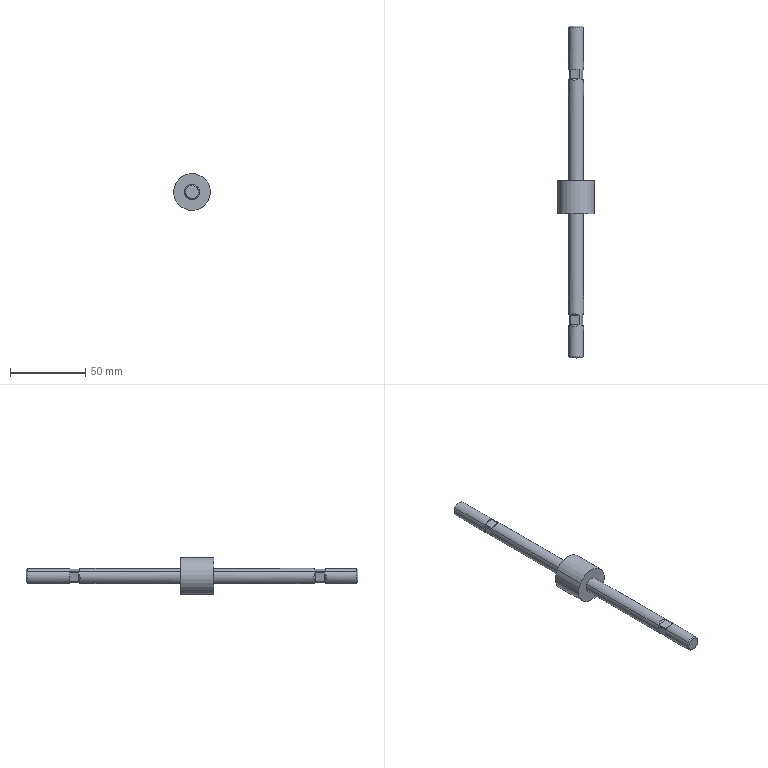Component | SolidWorks | MACJ25x25-10S-Rod-1_MACJ25x25-10S-Rod-1 | 1 solid | 38 faces | box 24.5 x 221 x 24.5 mm | volume 25761 mm3 | plane 28 | cylinder 6 | cone 4 | commonest cylinder face diameters 10 x4 24.5 x2
STEP:
#1=CARTESIAN_POINT('',(-0.3117,9.81,-6.329));
#2=VERTEX_POINT('',#1);
#3=CARTESIAN_POINT('',(-0.0297,9.81,-6.507));
#4=VERTEX_POINT('',#3);
#5=CARTESIAN_POINT('',(-0.1707,9.81,-6.418));
#6=DIRECTION('',(0.,-1.,-0.));
#7=DIRECTION('',(-0.846,0.,0.5333));
#8=AXIS2_PLACEMENT_3D('',#5,#6,#7);
#9=CIRCLE('',#8,0.1667);
#10=EDGE_CURVE('',#2,#4,#9,.T.);
#11=ORIENTED_EDGE('',*,*,#10,.T.);
#12=CARTESIAN_POINT('',(-0.00415,9.78,-6.523));
#13=VERTEX_POINT('',#12);
#14=CARTESIAN_POINT('',(-0.0297,9.81,-6.507));
#15=DIRECTION('',(0.5982,-0.7071,-0.3771));
#16=VECTOR('',#15,39.37);
#17=LINE('',#14,#16);
#18=EDGE_CURVE('',#4,#13,#17,.T.);
#19=ORIENTED_EDGE('',*,*,#18,.T.);
#20=CARTESIAN_POINT('',(-0.3372,9.78,-6.313));
#21=VERTEX_POINT('',#20);
#22=CARTESIAN_POINT('',(-0.1707,9.78,-6.418));
#23=DIRECTION('',(0.,-1.,-0.));
#24=DIRECTION('',(-0.846,0.,0.5333));
#25=AXIS2_PLACEMENT_3D('',#22,#23,#24);
#26=CIRCLE('',#25,0.1969);
#27=EDGE_CURVE('',#21,#13,#26,.T.);
#28=ORIENTED_EDGE('',*,*,#27,.F.);
#29=CARTESIAN_POINT('',(-0.3117,9.81,-6.329));
#30=DIRECTION('',(-0.5982,-0.7071,0.3771));
#31=VECTOR('',#30,39.37);
#32=LINE('',#29,#31);
#33=EDGE_CURVE('',#2,#21,#32,.T.);
#34=ORIENTED_EDGE('',*,*,#33,.F.);
#35=EDGE_LOOP('',(#11,#19,#28,#34));
#36=FACE_OUTER_BOUND('',#35,.T.);
#37=CARTESIAN_POINT('',(-0.1707,9.81,-6.418));
#38=DIRECTION('',(0.,-1.,-0.));
#39=DIRECTION('',(-0.846,0.,0.5333));
#40=AXIS2_PLACEMENT_3D('',#37,#38,#39);
#41=CONICAL_SURFACE('',#40,0.1667,0.7854);
#42=ADVANCED_FACE('',(#36),#41,.T.);
#43=CARTESIAN_POINT('',(-0.2981,8.432,-6.568));
#44=VERTEX_POINT('',#43);
#45=CARTESIAN_POINT('',(-0.2981,8.668,-6.568));
#46=VERTEX_POINT('',#45);
#47=CARTESIAN_POINT('',(-0.2981,9.81,-6.568));
#48=DIRECTION('',(-0.,1.,0.));
#49=VECTOR('',#48,39.37);
#50=LINE('',#47,#49);
#51=EDGE_CURVE('',#44,#46,#50,.T.);
#52=ORIENTED_EDGE('',*,*,#51,.T.);
#53=CARTESIAN_POINT('',(-0.3504,8.668,-6.338));
#54=VERTEX_POINT('',#53);
#55=CARTESIAN_POINT('',(-0.1707,8.668,-6.418));
#56=DIRECTION('',(-0.,1.,0.));
#57=DIRECTION('',(0.846,0.,-0.5333));
#58=AXIS2_PLACEMENT_3D('',#55,#56,#57);
#59=CIRCLE('',#58,0.1969);
#60=EDGE_CURVE('',#46,#54,#59,.T.);
#61=ORIENTED_EDGE('',*,*,#60,.T.);
#62=CARTESIAN_POINT('',(-0.3504,8.432,-6.338));
#63=VERTEX_POINT('',#62);
#64=CARTESIAN_POINT('',(-0.3504,9.81,-6.338));
#65=DIRECTION('',(0.,-1.,-0.));
#66=VECTOR('',#65,39.37);
#67=LINE('',#64,#66);
#68=EDGE_CURVE('',#54,#63,#67,.T.);
#69=ORIENTED_EDGE('',*,*,#68,.T.);
#70=CARTESIAN_POINT('',(-0.3504,8.432,-6.338));
#71=CARTESIAN_POINT('',(-0.3875,8.377,-6.42));
#72=CARTESIAN_POINT('',(-0.3674,8.377,-6.509));
#73=CARTESIAN_POINT('',(-0.2981,8.432,-6.568));
#74=(BOUNDED_CURVE()B_SPLINE_CURVE(3,(#70,#71,#72,#73),.UNSPECIFIED.,.F.,.T.)B_SPLINE_CURVE_WITH_KNOTS((4,4),(5.64,6.927),.UNSPECIFIED.)CURVE()GEOMETRIC_REPRESENTATION_ITEM()RATIONAL_B_SPLINE_CURVE((1.,0.8667,0.8667,1.))REPRESENTATION_ITEM(''));
#75=EDGE_CURVE('',#63,#44,#74,.T.);
#76=ORIENTED_EDGE('',*,*,#75,.T.);
#77=EDGE_LOOP('',(#52,#61,#69,#76));
#78=FACE_BOUND('',#77,.T.);
#79=CARTESIAN_POINT('',(-0.02067,8.432,-6.545));
#80=VERTEX_POINT('',#79);
#81=CARTESIAN_POINT('',(-0.02067,8.668,-6.545));
#82=VERTEX_POINT('',#81);
#83=CARTESIAN_POINT('',(-0.02067,9.81,-6.545));
#84=DIRECTION('',(-0.,1.,0.));
#85=VECTOR('',#84,39.37);
#86=LINE('',#83,#85);
#87=EDGE_CURVE('',#80,#82,#86,.T.);
#88=ORIENTED_EDGE('',*,*,#87,.T.);
#89=CARTESIAN_POINT('',(-0.251,8.668,-6.598));
#90=VERTEX_POINT('',#89);
#91=CARTESIAN_POINT('',(-0.1707,8.668,-6.418));
#92=DIRECTION('',(-0.,1.,0.));
#93=DIRECTION('',(0.846,0.,-0.5333));
#94=AXIS2_PLACEMENT_3D('',#91,#92,#93);
#95=CIRCLE('',#94,0.1969);
#96=EDGE_CURVE('',#82,#90,#95,.T.);
#97=ORIENTED_EDGE('',*,*,#96,.T.);
#98=CARTESIAN_POINT('',(-0.251,8.432,-6.598));
#99=VERTEX_POINT('',#98);
#100=CARTESIAN_POINT('',(-0.251,9.81,-6.598));
#101=DIRECTION('',(0.,-1.,-0.));
#102=VECTOR('',#101,39.37);
#103=LINE('',#100,#102);
#104=EDGE_CURVE('',#90,#99,#103,.T.);
#105=ORIENTED_EDGE('',*,*,#104,.T.);
#106=CARTESIAN_POINT('',(-0.251,8.432,-6.598));
#107=CARTESIAN_POINT('',(-0.1681,8.377,-6.635));
#108=CARTESIAN_POINT('',(-0.0795,8.377,-6.615));
#109=CARTESIAN_POINT('',(-0.02067,8.432,-6.545));
#110=(BOUNDED_CURVE()B_SPLINE_CURVE(3,(#106,#107,#108,#109),.UNSPECIFIED.,.F.,.F.)B_SPLINE_CURVE_WITH_KNOTS((4,4),(5.64,6.927),.UNSPECIFIED.)CURVE()GEOMETRIC_REPRESENTATION_ITEM()RATIONAL_B_SPLINE_CURVE((1.,0.8667,0.8667,1.))REPRESENTATION_ITEM(''));
#111=EDGE_CURVE('',#99,#80,#110,.T.);
#112=ORIENTED_EDGE('',*,*,#111,.T.);
#113=EDGE_LOOP('',(#88,#97,#105,#112));
#114=FACE_BOUND('',#113,.T.);
#115=ORIENTED_EDGE('',*,*,#27,.T.);
#116=CARTESIAN_POINT('',(-0.00415,5.755,-6.523));
#117=VERTEX_POINT('',#116);
#118=CARTESIAN_POINT('',(-0.00415,9.81,-6.523));
#119=DIRECTION('',(0.,-1.,-0.));
#120=VECTOR('',#119,39.37);
#121=LINE('',#118,#120);
#122=EDGE_CURVE('',#13,#117,#121,.T.);
#123=ORIENTED_EDGE('',*,*,#122,.T.);
#124=CARTESIAN_POINT('',(-0.3372,5.755,-6.313));
#125=VERTEX_POINT('',#124);
#126=CARTESIAN_POINT('',(-0.1707,5.755,-6.418));
#127=DIRECTION('',(0.,-1.,-0.));
#128=DIRECTION('',(-0.846,0.,0.5333));
#129=AXIS2_PLACEMENT_3D('',#126,#127,#128);
#130=CIRCLE('',#129,0.1969);
#131=EDGE_CURVE('',#125,#117,#130,.T.);
#132=ORIENTED_EDGE('',*,*,#131,.F.);
#133=CARTESIAN_POINT('',(-0.3372,9.81,-6.313));
#134=DIRECTION('',(0.,-1.,-0.));
#135=VECTOR('',#134,39.37);
#136=LINE('',#133,#135);
#137=EDGE_CURVE('',#21,#125,#136,.T.);
#138=ORIENTED_EDGE('',*,*,#137,.F.);
#139=EDGE_LOOP('',(#115,#123,#132,#138));
#140=FACE_OUTER_BOUND('',#139,.T.);
#141=CARTESIAN_POINT('',(-0.1707,9.81,-6.418));
#142=DIRECTION('',(0.,-1.,-0.));
#143=DIRECTION('',(-0.846,0.,0.5333));
#144=AXIS2_PLACEMENT_3D('',#141,#142,#143);
#145=CYLINDRICAL_SURFACE('',#144,0.1969);
#146=ADVANCED_FACE('',(#78,#114,#140),#145,.T.);
#147=CARTESIAN_POINT('',(-0.5787,5.755,-6.161));
#148=VERTEX_POINT('',#147);
#149=CARTESIAN_POINT('',(0.2373,5.755,-6.675));
#150=VERTEX_POINT('',#149);
#151=CARTESIAN_POINT('',(-0.1707,5.755,-6.418));
#152=DIRECTION('',(0.,-1.,-0.));
#153=DIRECTION('',(-0.846,0.,0.5333));
#154=AXIS2_PLACEMENT_3D('',#151,#152,#153);
#155=CIRCLE('',#154,0.4823);
#156=EDGE_CURVE('',#148,#150,#155,.T.);
#157=ORIENTED_EDGE('',*,*,#156,.T.);
#158=CARTESIAN_POINT('',(0.2373,4.889,-6.675));
#159=VERTEX_POINT('',#158);
#160=CARTESIAN_POINT('',(0.2373,9.81,-6.675));
#161=DIRECTION('',(0.,-1.,-0.));
#162=VECTOR('',#161,39.37);
#163=LINE('',#160,#162);
#164=EDGE_CURVE('',#150,#159,#163,.T.);
#165=ORIENTED_EDGE('',*,*,#164,.T.);
#166=CARTESIAN_POINT('',(-0.5787,4.889,-6.161));
#167=VERTEX_POINT('',#166);
#168=CARTESIAN_POINT('',(-0.1707,4.889,-6.418));
#169=DIRECTION('',(0.,-1.,-0.));
#170=DIRECTION('',(-0.846,0.,0.5333));
#171=AXIS2_PLACEMENT_3D('',#168,#169,#170);
#172=CIRCLE('',#171,0.4823);
#173=EDGE_CURVE('',#167,#159,#172,.T.);
#174=ORIENTED_EDGE('',*,*,#173,.F.);
#175=CARTESIAN_POINT('',(-0.5787,9.81,-6.161));
#176=DIRECTION('',(0.,-1.,-0.));
#177=VECTOR('',#176,39.37);
#178=LINE('',#175,#177);
#179=EDGE_CURVE('',#148,#167,#178,.T.);
#180=ORIENTED_EDGE('',*,*,#179,.F.);
#181=EDGE_LOOP('',(#157,#165,#174,#180));
#182=FACE_OUTER_BOUND('',#181,.T.);
#183=CARTESIAN_POINT('',(-0.1707,9.81,-6.418));
#184=DIRECTION('',(0.,-1.,-0.));
#185=DIRECTION('',(-0.846,0.,0.5333));
#186=AXIS2_PLACEMENT_3D('',#183,#184,#185);
#187=CYLINDRICAL_SURFACE('',#186,0.4823);
#188=ADVANCED_FACE('',(#182),#187,.T.);
#189=CARTESIAN_POINT('',(-0.2981,1.975,-6.568));
#190=VERTEX_POINT('',#189);
#191=CARTESIAN_POINT('',(-0.2981,2.227,-6.568));
#192=VERTEX_POINT('',#191);
#193=CARTESIAN_POINT('',(-0.2981,9.81,-6.568));
#194=DIRECTION('',(-0.,1.,0.));
#195=VECTOR('',#194,39.37);
#196=LINE('',#193,#195);
#197=EDGE_CURVE('',#190,#192,#196,.T.);
#198=ORIENTED_EDGE('',*,*,#197,.T.);
#199=CARTESIAN_POINT('',(-0.3504,2.227,-6.338));
#200=VERTEX_POINT('',#199);
#201=CARTESIAN_POINT('',(-0.2981,2.227,-6.568));
#202=CARTESIAN_POINT('',(-0.3674,2.282,-6.509));
#203=CARTESIAN_POINT('',(-0.3875,2.282,-6.42));
#204=CARTESIAN_POINT('',(-0.3504,2.227,-6.338));
#205=(BOUNDED_CURVE()B_SPLINE_CURVE(3,(#201,#202,#203,#204),.UNSPECIFIED.,.F.,.T.)B_SPLINE_CURVE_WITH_KNOTS((4,4),(2.498,3.785),.UNSPECIFIED.)CURVE()GEOMETRIC_REPRESENTATION_ITEM()RATIONAL_B_SPLINE_CURVE((1.,0.8667,0.8667,1.))REPRESENTATION_ITEM(''));
#206=EDGE_CURVE('',#192,#200,#205,.T.);
#207=ORIENTED_EDGE('',*,*,#206,.T.);
#208=CARTESIAN_POINT('',(-0.3504,1.975,-6.338));
#209=VERTEX_POINT('',#208);
#210=CARTESIAN_POINT('',(-0.3504,9.81,-6.338));
#211=DIRECTION('',(0.,-1.,-0.));
#212=VECTOR('',#211,39.37);
#213=LINE('',#210,#212);
#214=EDGE_CURVE('',#200,#209,#213,.T.);
#215=ORIENTED_EDGE('',*,*,#214,.T.);
#216=CARTESIAN_POINT('',(-0.3504,1.975,-6.338));
#217=CARTESIAN_POINT('',(-0.3875,1.921,-6.42));
#218=CARTESIAN_POINT('',(-0.3674,1.921,-6.509));
#219=CARTESIAN_POINT('',(-0.2981,1.975,-6.568));
#220=(BOUNDED_CURVE()B_SPLINE_CURVE(3,(#216,#217,#218,#219),.UNSPECIFIED.,.F.,.F.)B_SPLINE_CURVE_WITH_KNOTS((4,4),(5.64,6.927),.UNSPECIFIED.)CURVE()GEOMETRIC_REPRESENTATION_ITEM()RATIONAL_B_SPLINE_CURVE((1.,0.8667,0.8667,1.))REPRESENTATION_ITEM(''));
#221=EDGE_CURVE('',#209,#190,#220,.T.);
#222=ORIENTED_EDGE('',*,*,#221,.T.);
#223=EDGE_LOOP('',(#198,#207,#215,#222));
#224=FACE_BOUND('',#223,.T.);
#225=CARTESIAN_POINT('',(-0.02067,1.975,-6.545));
#226=VERTEX_POINT('',#225);
#227=CARTESIAN_POINT('',(-0.02067,2.227,-6.545));
#228=VERTEX_POINT('',#227);
#229=CARTESIAN_POINT('',(-0.02067,9.81,-6.545));
#230=DIRECTION('',(-0.,1.,0.));
#231=VECTOR('',#230,39.37);
#232=LINE('',#229,#231);
#233=EDGE_CURVE('',#226,#228,#232,.T.);
#234=ORIENTED_EDGE('',*,*,#233,.T.);
#235=CARTESIAN_POINT('',(-0.251,2.227,-6.598));
#236=VERTEX_POINT('',#235);
#237=CARTESIAN_POINT('',(-0.02067,2.227,-6.545));
#238=CARTESIAN_POINT('',(-0.0795,2.282,-6.615));
#239=CARTESIAN_POINT('',(-0.1681,2.282,-6.635));
#240=CARTESIAN_POINT('',(-0.251,2.227,-6.598));
#241=(BOUNDED_CURVE()B_SPLINE_CURVE(3,(#237,#238,#239,#240),.UNSPECIFIED.,.F.,.T.)B_SPLINE_CURVE_WITH_KNOTS((4,4),(2.498,3.785),.UNSPECIFIED.)CURVE()GEOMETRIC_REPRESENTATION_ITEM()RATIONAL_B_SPLINE_CURVE((1.,0.8667,0.8667,1.))REPRESENTATION_ITEM(''));
#242=EDGE_CURVE('',#228,#236,#241,.T.);
#243=ORIENTED_EDGE('',*,*,#242,.T.);
#244=CARTESIAN_POINT('',(-0.251,1.975,-6.598));
#245=VERTEX_POINT('',#244);
#246=CARTESIAN_POINT('',(-0.251,9.81,-6.598));
#247=DIRECTION('',(0.,-1.,-0.));
#248=VECTOR('',#247,39.37);
#249=LINE('',#246,#248);
#250=EDGE_CURVE('',#236,#245,#249,.T.);
#251=ORIENTED_EDGE('',*,*,#250,.T.);
#252=CARTESIAN_POINT('',(-0.251,1.975,-6.598));
#253=CARTESIAN_POINT('',(-0.1681,1.921,-6.635));
#254=CARTESIAN_POINT('',(-0.0795,1.921,-6.615));
#255=CARTESIAN_POINT('',(-0.02067,1.975,-6.545));
#256=(BOUNDED_CURVE()B_SPLINE_CURVE(3,(#252,#253,#254,#255),.UNSPECIFIED.,.F.,.T.)B_SPLINE_CURVE_WITH_KNOTS((4,4),(5.64,6.927),.UNSPECIFIED.)CURVE()GEOMETRIC_REPRESENTATION_ITEM()RATIONAL_B_SPLINE_CURVE((1.,0.8667,0.8667,1.))REPRESENTATION_ITEM(''));
#257=EDGE_CURVE('',#245,#226,#256,.T.);
#258=ORIENTED_EDGE('',*,*,#257,.T.);
#259=EDGE_LOOP('',(#234,#243,#251,#258));
#260=FACE_BOUND('',#259,.T.);
#261=CARTESIAN_POINT('',(-0.3372,4.889,-6.313));
#262=VERTEX_POINT('',#261);
#263=CARTESIAN_POINT('',(-0.00415,4.889,-6.523));
#264=VERTEX_POINT('',#263);
#265=CARTESIAN_POINT('',(-0.1707,4.889,-6.418));
#266=DIRECTION('',(0.,-1.,-0.));
#267=DIRECTION('',(-0.846,0.,0.5333));
#268=AXIS2_PLACEMENT_3D('',#265,#266,#267);
#269=CIRCLE('',#268,0.1969);
#270=EDGE_CURVE('',#262,#264,#269,.T.);
#271=ORIENTED_EDGE('',*,*,#270,.T.);
#272=CARTESIAN_POINT('',(-0.00415,1.139,-6.523));
#273=VERTEX_POINT('',#272);
#274=CARTESIAN_POINT('',(-0.00415,9.81,-6.523));
#275=DIRECTION('',(0.,-1.,-0.));
#276=VECTOR('',#275,39.37);
#277=LINE('',#274,#276);
#278=EDGE_CURVE('',#264,#273,#277,.T.);
#279=ORIENTED_EDGE('',*,*,#278,.T.);
#280=CARTESIAN_POINT('',(-0.3372,1.139,-6.313));
#281=VERTEX_POINT('',#280);
#282=CARTESIAN_POINT('',(-0.1707,1.139,-6.418));
#283=DIRECTION('',(0.,-1.,-0.));
#284=DIRECTION('',(-0.846,0.,0.5333));
#285=AXIS2_PLACEMENT_3D('',#282,#283,#284);
#286=CIRCLE('',#285,0.1969);
#287=EDGE_CURVE('',#281,#273,#286,.T.);
#288=ORIENTED_EDGE('',*,*,#287,.F.);
#289=CARTESIAN_POINT('',(-0.3372,9.81,-6.313));
#290=DIRECTION('',(0.,-1.,-0.));
#291=VECTOR('',#290,39.37);
#292=LINE('',#289,#291);
#293=EDGE_CURVE('',#262,#281,#292,.T.);
#294=ORIENTED_EDGE('',*,*,#293,.F.);
#295=EDGE_LOOP('',(#271,#279,#288,#294));
#296=FACE_OUTER_BOUND('',#295,.T.);
#297=CARTESIAN_POINT('',(-0.1707,9.81,-6.418));
#298=DIRECTION('',(0.,-1.,-0.));
#299=DIRECTION('',(-0.846,0.,0.5333));
#300=AXIS2_PLACEMENT_3D('',#297,#298,#299);
#301=CYLINDRICAL_SURFACE('',#300,0.1969);
#302=ADVANCED_FACE('',(#224,#260,#296),#301,.T.);
#303=CARTESIAN_POINT('',(-0.3117,1.109,-6.329));
#304=VERTEX_POINT('',#303);
#305=CARTESIAN_POINT('',(-0.0297,1.109,-6.507));
#306=VERTEX_POINT('',#305);
#307=CARTESIAN_POINT('',(-0.1707,1.109,-6.418));
#308=DIRECTION('',(0.,-1.,-0.));
#309=DIRECTION('',(-0.846,0.,0.5333));
#310=AXIS2_PLACEMENT_3D('',#307,#308,#309);
#311=CIRCLE('',#310,0.1667);
#312=EDGE_CURVE('',#304,#306,#311,.T.);
#313=ORIENTED_EDGE('',*,*,#312,.F.);
#314=CARTESIAN_POINT('',(-0.3372,1.139,-6.313));
#315=DIRECTION('',(-0.5982,0.7071,0.3771));
#316=VECTOR('',#315,39.37);
#317=LINE('',#314,#316);
#318=EDGE_CURVE('',#304,#281,#317,.T.);
#319=ORIENTED_EDGE('',*,*,#318,.T.);
#320=ORIENTED_EDGE('',*,*,#287,.T.);
#321=CARTESIAN_POINT('',(-0.00415,1.139,-6.523));
#322=DIRECTION('',(0.5982,0.7071,-0.3771));
#323=VECTOR('',#322,39.37);
#324=LINE('',#321,#323);
#325=EDGE_CURVE('',#306,#273,#324,.T.);
#326=ORIENTED_EDGE('',*,*,#325,.F.);
#327=EDGE_LOOP('',(#313,#319,#320,#326));
#328=FACE_OUTER_BOUND('',#327,.T.);
#329=CARTESIAN_POINT('',(-0.1707,1.139,-6.418));
#330=DIRECTION('',(-0.,1.,0.));
#331=DIRECTION('',(0.846,0.,-0.5333));
#332=AXIS2_PLACEMENT_3D('',#329,#330,#331);
#333=CONICAL_SURFACE('',#332,0.1969,0.7854);
#334=ADVANCED_FACE('',(#328),#333,.T.);
#335=CARTESIAN_POINT('',(-0.1707,1.109,-6.418));
#336=DIRECTION('',(0.,-1.,-0.));
#337=DIRECTION('',(-0.846,0.,0.5333));
#338=AXIS2_PLACEMENT_3D('',#335,#336,#337);
#339=CIRCLE('',#338,0.1667);
#340=EDGE_CURVE('',#306,#304,#339,.T.);
#341=ORIENTED_EDGE('',*,*,#340,.T.);
#342=ORIENTED_EDGE('',*,*,#312,.T.);
#343=EDGE_LOOP('',(#341,#342));
#344=FACE_OUTER_BOUND('',#343,.T.);
#345=CARTESIAN_POINT('',(-0.1707,1.109,-6.418));
#346=DIRECTION('',(-0.,1.,0.));
#347=DIRECTION('',(0.846,0.,-0.5333));
#348=AXIS2_PLACEMENT_3D('',#345,#346,#347);
#349=PLANE('',#348);
#350=ADVANCED_FACE('',(#344),#349,.F.);
#351=ORIENTED_EDGE('',*,*,#318,.F.);
#352=ORIENTED_EDGE('',*,*,#340,.F.);
#353=ORIENTED_EDGE('',*,*,#325,.T.);
#354=CARTESIAN_POINT('',(-0.1707,1.139,-6.418));
#355=DIRECTION('',(0.,-1.,-0.));
#356=DIRECTION('',(-0.846,0.,0.5333));
#357=AXIS2_PLACEMENT_3D('',#354,#355,#356);
#358=CIRCLE('',#357,0.1969);
#359=EDGE_CURVE('',#273,#281,#358,.T.);
#360=ORIENTED_EDGE('',*,*,#359,.T.);
#361=EDGE_LOOP('',(#351,#352,#353,#360));
#362=FACE_OUTER_BOUND('',#361,.T.);
#363=CARTESIAN_POINT('',(-0.1707,1.139,-6.418));
#364=DIRECTION('',(-0.,1.,0.));
#365=DIRECTION('',(0.846,0.,-0.5333));
#366=AXIS2_PLACEMENT_3D('',#363,#364,#365);
#367=CONICAL_SURFACE('',#366,0.1969,0.7854);
#368=ADVANCED_FACE('',(#362),#367,.T.);
#369=ORIENTED_EDGE('',*,*,#278,.F.);
#370=CARTESIAN_POINT('',(-0.1707,4.889,-6.418));
#371=DIRECTION('',(0.,-1.,-0.));
#372=DIRECTION('',(-0.846,0.,0.5333));
#373=AXIS2_PLACEMENT_3D('',#370,#371,#372);
#374=CIRCLE('',#373,0.1969);
#375=EDGE_CURVE('',#264,#262,#374,.T.);
#376=ORIENTED_EDGE('',*,*,#375,.T.);
#377=ORIENTED_EDGE('',*,*,#293,.T.);
#378=ORIENTED_EDGE('',*,*,#359,.F.);
#379=EDGE_LOOP('',(#369,#376,#377,#378));
#380=FACE_OUTER_BOUND('',#379,.T.);
#381=CARTESIAN_POINT('',(-0.09031,2.227,-6.238));
#382=VERTEX_POINT('',#381);
#383=CARTESIAN_POINT('',(-0.09031,1.975,-6.238));
#384=VERTEX_POINT('',#383);
#385=CARTESIAN_POINT('',(-0.09031,9.81,-6.238));
#386=DIRECTION('',(0.,-1.,-0.));
#387=VECTOR('',#386,39.37);
#388=LINE('',#385,#387);
#389=EDGE_CURVE('',#382,#384,#388,.T.);
#390=ORIENTED_EDGE('',*,*,#389,.T.);
#391=CARTESIAN_POINT('',(-0.3207,1.975,-6.29));
#392=VERTEX_POINT('',#391);
#393=CARTESIAN_POINT('',(-0.09031,1.975,-6.238));
#394=CARTESIAN_POINT('',(-0.1732,1.921,-6.201));
#395=CARTESIAN_POINT('',(-0.2619,1.921,-6.221));
#396=CARTESIAN_POINT('',(-0.3207,1.975,-6.29));
#397=(BOUNDED_CURVE()B_SPLINE_CURVE(3,(#393,#394,#395,#396),.UNSPECIFIED.,.F.,.F.)B_SPLINE_CURVE_WITH_KNOTS((4,4),(5.64,6.927),.UNSPECIFIED.)CURVE()GEOMETRIC_REPRESENTATION_ITEM()RATIONAL_B_SPLINE_CURVE((1.,0.8667,0.8667,1.))REPRESENTATION_ITEM(''));
#398=EDGE_CURVE('',#384,#392,#397,.T.);
#399=ORIENTED_EDGE('',*,*,#398,.T.);
#400=CARTESIAN_POINT('',(-0.3207,2.227,-6.29));
#401=VERTEX_POINT('',#400);
#402=CARTESIAN_POINT('',(-0.3207,9.81,-6.29));
#403=DIRECTION('',(-0.,1.,0.));
#404=VECTOR('',#403,39.37);
#405=LINE('',#402,#404);
#406=EDGE_CURVE('',#392,#401,#405,.T.);
#407=ORIENTED_EDGE('',*,*,#406,.T.);
#408=CARTESIAN_POINT('',(-0.3207,2.227,-6.29));
#409=CARTESIAN_POINT('',(-0.2619,2.282,-6.221));
#410=CARTESIAN_POINT('',(-0.1732,2.282,-6.201));
#411=CARTESIAN_POINT('',(-0.09031,2.227,-6.238));
#412=(BOUNDED_CURVE()B_SPLINE_CURVE(3,(#408,#409,#410,#411),.UNSPECIFIED.,.F.,.F.)B_SPLINE_CURVE_WITH_KNOTS((4,4),(2.498,3.785),.UNSPECIFIED.)CURVE()GEOMETRIC_REPRESENTATION_ITEM()RATIONAL_B_SPLINE_CURVE((1.,0.8667,0.8667,1.))REPRESENTATION_ITEM(''));
#413=EDGE_CURVE('',#401,#382,#412,.T.);
#414=ORIENTED_EDGE('',*,*,#413,.T.);
#415=EDGE_LOOP('',(#390,#399,#407,#414));
#416=FACE_BOUND('',#415,.T.);
#417=CARTESIAN_POINT('',(0.009021,2.227,-6.498));
#418=VERTEX_POINT('',#417);
#419=CARTESIAN_POINT('',(0.009021,1.975,-6.498));
#420=VERTEX_POINT('',#419);
#421=CARTESIAN_POINT('',(0.009021,9.81,-6.498));
#422=DIRECTION('',(0.,-1.,-0.));
#423=VECTOR('',#422,39.37);
#424=LINE('',#421,#423);
#425=EDGE_CURVE('',#418,#420,#424,.T.);
#426=ORIENTED_EDGE('',*,*,#425,.T.);
#427=CARTESIAN_POINT('',(-0.04321,1.975,-6.268));
#428=VERTEX_POINT('',#427);
#429=CARTESIAN_POINT('',(0.009021,1.975,-6.498));
#430=CARTESIAN_POINT('',(0.04611,1.921,-6.415));
#431=CARTESIAN_POINT('',(0.02603,1.921,-6.327));
#432=CARTESIAN_POINT('',(-0.04321,1.975,-6.268));
#433=(BOUNDED_CURVE()B_SPLINE_CURVE(3,(#429,#430,#431,#432),.UNSPECIFIED.,.F.,.F.)B_SPLINE_CURVE_WITH_KNOTS((4,4),(5.64,6.927),.UNSPECIFIED.)CURVE()GEOMETRIC_REPRESENTATION_ITEM()RATIONAL_B_SPLINE_CURVE((1.,0.8667,0.8667,1.))REPRESENTATION_ITEM(''));
#434=EDGE_CURVE('',#420,#428,#433,.T.);
#435=ORIENTED_EDGE('',*,*,#434,.T.);
#436=CARTESIAN_POINT('',(-0.04321,2.227,-6.268));
#437=VERTEX_POINT('',#436);
#438=CARTESIAN_POINT('',(-0.04321,9.81,-6.268));
#439=DIRECTION('',(-0.,1.,0.));
#440=VECTOR('',#439,39.37);
#441=LINE('',#438,#440);
#442=EDGE_CURVE('',#428,#437,#441,.T.);
#443=ORIENTED_EDGE('',*,*,#442,.T.);
#444=CARTESIAN_POINT('',(-0.04321,2.227,-6.268));
#445=CARTESIAN_POINT('',(0.02603,2.282,-6.327));
#446=CARTESIAN_POINT('',(0.04611,2.282,-6.415));
#447=CARTESIAN_POINT('',(0.009021,2.227,-6.498));
#448=(BOUNDED_CURVE()B_SPLINE_CURVE(3,(#444,#445,#446,#447),.UNSPECIFIED.,.F.,.F.)B_SPLINE_CURVE_WITH_KNOTS((4,4),(2.498,3.785),.UNSPECIFIED.)CURVE()GEOMETRIC_REPRESENTATION_ITEM()RATIONAL_B_SPLINE_CURVE((1.,0.8667,0.8667,1.))REPRESENTATION_ITEM(''));
#449=EDGE_CURVE('',#437,#418,#448,.T.);
#450=ORIENTED_EDGE('',*,*,#449,.T.);
#451=EDGE_LOOP('',(#426,#435,#443,#450));
#452=FACE_BOUND('',#451,.T.);
#453=CARTESIAN_POINT('',(-0.1707,9.81,-6.418));
#454=DIRECTION('',(0.,-1.,-0.));
#455=DIRECTION('',(-0.846,0.,0.5333));
#456=AXIS2_PLACEMENT_3D('',#453,#454,#455);
#457=CYLINDRICAL_SURFACE('',#456,0.1969);
#458=ADVANCED_FACE('',(#380,#416,#452),#457,.T.);
#459=ORIENTED_EDGE('',*,*,#270,.F.);
#460=ORIENTED_EDGE('',*,*,#375,.F.);
#461=EDGE_LOOP('',(#459,#460));
#462=FACE_BOUND('',#461,.T.);
#463=ORIENTED_EDGE('',*,*,#173,.T.);
#464=CARTESIAN_POINT('',(-0.1707,4.889,-6.418));
#465=DIRECTION('',(0.,-1.,-0.));
#466=DIRECTION('',(-0.846,0.,0.5333));
#467=AXIS2_PLACEMENT_3D('',#464,#465,#466);
#468=CIRCLE('',#467,0.4823);
#469=EDGE_CURVE('',#159,#167,#468,.T.);
#470=ORIENTED_EDGE('',*,*,#469,.T.);
#471=EDGE_LOOP('',(#463,#470));
#472=FACE_OUTER_BOUND('',#471,.T.);
#473=CARTESIAN_POINT('',(-0.2756,4.889,-6.584));
#474=DIRECTION('',(-0.,1.,0.));
#475=DIRECTION('',(0.846,0.,-0.5333));
#476=AXIS2_PLACEMENT_3D('',#473,#474,#475);
#477=PLANE('',#476);
#478=ADVANCED_FACE('',(#462,#472),#477,.F.);
#479=ORIENTED_EDGE('',*,*,#164,.F.);
#480=CARTESIAN_POINT('',(-0.1707,5.755,-6.418));
#481=DIRECTION('',(0.,-1.,-0.));
#482=DIRECTION('',(-0.846,0.,0.5333));
#483=AXIS2_PLACEMENT_3D('',#480,#481,#482);
#484=CIRCLE('',#483,0.4823);
#485=EDGE_CURVE('',#150,#148,#484,.T.);
#486=ORIENTED_EDGE('',*,*,#485,.T.);
#487=ORIENTED_EDGE('',*,*,#179,.T.);
#488=ORIENTED_EDGE('',*,*,#469,.F.);
#489=EDGE_LOOP('',(#479,#486,#487,#488));
#490=FACE_OUTER_BOUND('',#489,.T.);
#491=CARTESIAN_POINT('',(-0.1707,9.81,-6.418));
#492=DIRECTION('',(0.,-1.,-0.));
#493=DIRECTION('',(-0.846,0.,0.5333));
#494=AXIS2_PLACEMENT_3D('',#491,#492,#493);
#495=CYLINDRICAL_SURFACE('',#494,0.4823);
#496=ADVANCED_FACE('',(#490),#495,.T.);
#497=ORIENTED_EDGE('',*,*,#156,.F.);
#498=ORIENTED_EDGE('',*,*,#485,.F.);
#499=EDGE_LOOP('',(#497,#498));
#500=FACE_OUTER_BOUND('',#499,.T.);
#501=ORIENTED_EDGE('',*,*,#131,.T.);
#502=CARTESIAN_POINT('',(-0.1707,5.755,-6.418));
#503=DIRECTION('',(0.,-1.,-0.));
#504=DIRECTION('',(-0.846,0.,0.5333));
#505=AXIS2_PLACEMENT_3D('',#502,#503,#504);
#506=CIRCLE('',#505,0.1969);
#507=EDGE_CURVE('',#117,#125,#506,.T.);
#508=ORIENTED_EDGE('',*,*,#507,.T.);
#509=EDGE_LOOP('',(#501,#508));
#510=FACE_BOUND('',#509,.T.);
#511=CARTESIAN_POINT('',(-0.4279,5.755,-6.826));
#512=DIRECTION('',(0.,-1.,-0.));
#513=DIRECTION('',(-0.846,-0.,0.5333));
#514=AXIS2_PLACEMENT_3D('',#511,#512,#513);
#515=PLANE('',#514);
#516=ADVANCED_FACE('',(#500,#510),#515,.F.);
#517=ORIENTED_EDGE('',*,*,#122,.F.);
#518=CARTESIAN_POINT('',(-0.1707,9.78,-6.418));
#519=DIRECTION('',(0.,-1.,-0.));
#520=DIRECTION('',(-0.846,0.,0.5333));
#521=AXIS2_PLACEMENT_3D('',#518,#519,#520);
#522=CIRCLE('',#521,0.1969);
#523=EDGE_CURVE('',#13,#21,#522,.T.);
#524=ORIENTED_EDGE('',*,*,#523,.T.);
#525=ORIENTED_EDGE('',*,*,#137,.T.);
#526=ORIENTED_EDGE('',*,*,#507,.F.);
#527=EDGE_LOOP('',(#517,#524,#525,#526));
#528=FACE_OUTER_BOUND('',#527,.T.);
#529=CARTESIAN_POINT('',(-0.09031,8.668,-6.238));
#530=VERTEX_POINT('',#529);
#531=CARTESIAN_POINT('',(-0.09031,8.432,-6.238));
#532=VERTEX_POINT('',#531);
#533=CARTESIAN_POINT('',(-0.09031,9.81,-6.238));
#534=DIRECTION('',(0.,-1.,-0.));
#535=VECTOR('',#534,39.37);
#536=LINE('',#533,#535);
#537=EDGE_CURVE('',#530,#532,#536,.T.);
#538=ORIENTED_EDGE('',*,*,#537,.T.);
#539=CARTESIAN_POINT('',(-0.3207,8.432,-6.29));
#540=VERTEX_POINT('',#539);
#541=CARTESIAN_POINT('',(-0.09031,8.432,-6.238));
#542=CARTESIAN_POINT('',(-0.1732,8.377,-6.201));
#543=CARTESIAN_POINT('',(-0.2619,8.377,-6.221));
#544=CARTESIAN_POINT('',(-0.3207,8.432,-6.29));
#545=(BOUNDED_CURVE()B_SPLINE_CURVE(3,(#541,#542,#543,#544),.UNSPECIFIED.,.F.,.F.)B_SPLINE_CURVE_WITH_KNOTS((4,4),(5.64,6.927),.UNSPECIFIED.)CURVE()GEOMETRIC_REPRESENTATION_ITEM()RATIONAL_B_SPLINE_CURVE((1.,0.8667,0.8667,1.))REPRESENTATION_ITEM(''));
#546=EDGE_CURVE('',#532,#540,#545,.T.);
#547=ORIENTED_EDGE('',*,*,#546,.T.);
#548=CARTESIAN_POINT('',(-0.3207,8.668,-6.29));
#549=VERTEX_POINT('',#548);
#550=CARTESIAN_POINT('',(-0.3207,9.81,-6.29));
#551=DIRECTION('',(-0.,1.,0.));
#552=VECTOR('',#551,39.37);
#553=LINE('',#550,#552);
#554=EDGE_CURVE('',#540,#549,#553,.T.);
#555=ORIENTED_EDGE('',*,*,#554,.T.);
#556=CARTESIAN_POINT('',(-0.1707,8.668,-6.418));
#557=DIRECTION('',(-0.,1.,0.));
#558=DIRECTION('',(0.846,0.,-0.5333));
#559=AXIS2_PLACEMENT_3D('',#556,#557,#558);
#560=CIRCLE('',#559,0.1969);
#561=EDGE_CURVE('',#549,#530,#560,.T.);
#562=ORIENTED_EDGE('',*,*,#561,.T.);
#563=EDGE_LOOP('',(#538,#547,#555,#562));
#564=FACE_BOUND('',#563,.T.);
#565=CARTESIAN_POINT('',(0.009021,8.668,-6.498));
#566=VERTEX_POINT('',#565);
#567=CARTESIAN_POINT('',(0.009021,8.432,-6.498));
#568=VERTEX_POINT('',#567);
#569=CARTESIAN_POINT('',(0.009021,9.81,-6.498));
#570=DIRECTION('',(0.,-1.,-0.));
#571=VECTOR('',#570,39.37);
#572=LINE('',#569,#571);
#573=EDGE_CURVE('',#566,#568,#572,.T.);
#574=ORIENTED_EDGE('',*,*,#573,.T.);
#575=CARTESIAN_POINT('',(-0.04321,8.432,-6.268));
#576=VERTEX_POINT('',#575);
#577=CARTESIAN_POINT('',(0.009021,8.432,-6.498));
#578=CARTESIAN_POINT('',(0.04611,8.377,-6.415));
#579=CARTESIAN_POINT('',(0.02603,8.377,-6.327));
#580=CARTESIAN_POINT('',(-0.04321,8.432,-6.268));
#581=(BOUNDED_CURVE()B_SPLINE_CURVE(3,(#577,#578,#579,#580),.UNSPECIFIED.,.F.,.F.)B_SPLINE_CURVE_WITH_KNOTS((4,4),(5.64,6.927),.UNSPECIFIED.)CURVE()GEOMETRIC_REPRESENTATION_ITEM()RATIONAL_B_SPLINE_CURVE((1.,0.8667,0.8667,1.))REPRESENTATION_ITEM(''));
#582=EDGE_CURVE('',#568,#576,#581,.T.);
#583=ORIENTED_EDGE('',*,*,#582,.T.);
#584=CARTESIAN_POINT('',(-0.04321,8.668,-6.268));
#585=VERTEX_POINT('',#584);
#586=CARTESIAN_POINT('',(-0.04321,9.81,-6.268));
#587=DIRECTION('',(-0.,1.,0.));
#588=VECTOR('',#587,39.37);
#589=LINE('',#586,#588);
#590=EDGE_CURVE('',#576,#585,#589,.T.);
#591=ORIENTED_EDGE('',*,*,#590,.T.);
#592=CARTESIAN_POINT('',(-0.1707,8.668,-6.418));
#593=DIRECTION('',(-0.,1.,0.));
#594=DIRECTION('',(0.846,0.,-0.5333));
#595=AXIS2_PLACEMENT_3D('',#592,#593,#594);
#596=CIRCLE('',#595,0.1969);
#597=EDGE_CURVE('',#585,#566,#596,.T.);
#598=ORIENTED_EDGE('',*,*,#597,.T.);
#599=EDGE_LOOP('',(#574,#583,#591,#598));
#600=FACE_BOUND('',#599,.T.);
#601=CARTESIAN_POINT('',(-0.1707,9.81,-6.418));
#602=DIRECTION('',(0.,-1.,-0.));
#603=DIRECTION('',(-0.846,0.,0.5333));
#604=AXIS2_PLACEMENT_3D('',#601,#602,#603);
#605=CYLINDRICAL_SURFACE('',#604,0.1969);
#606=ADVANCED_FACE('',(#528,#564,#600),#605,.T.);
#607=ORIENTED_EDGE('',*,*,#18,.F.);
#608=CARTESIAN_POINT('',(-0.1707,9.81,-6.418));
#609=DIRECTION('',(0.,-1.,-0.));
#610=DIRECTION('',(-0.846,0.,0.5333));
#611=AXIS2_PLACEMENT_3D('',#608,#609,#610);
#612=CIRCLE('',#611,0.1667);
#613=EDGE_CURVE('',#4,#2,#612,.T.);
#614=ORIENTED_EDGE('',*,*,#613,.T.);
#615=ORIENTED_EDGE('',*,*,#33,.T.);
#616=ORIENTED_EDGE('',*,*,#523,.F.);
#617=EDGE_LOOP('',(#607,#614,#615,#616));
#618=FACE_OUTER_BOUND('',#617,.T.);
#619=CARTESIAN_POINT('',(-0.1707,9.81,-6.418));
#620=DIRECTION('',(0.,-1.,-0.));
#621=DIRECTION('',(-0.846,0.,0.5333));
#622=AXIS2_PLACEMENT_3D('',#619,#620,#621);
#623=CONICAL_SURFACE('',#622,0.1667,0.7854);
#624=ADVANCED_FACE('',(#618),#623,.T.);
#625=ORIENTED_EDGE('',*,*,#10,.F.);
#626=ORIENTED_EDGE('',*,*,#613,.F.);
#627=EDGE_LOOP('',(#625,#626));
#628=FACE_OUTER_BOUND('',#627,.T.);
#629=CARTESIAN_POINT('',(-0.2595,9.81,-6.559));
#630=DIRECTION('',(0.,-1.,-0.));
#631=DIRECTION('',(-0.846,-0.,0.5333));
#632=AXIS2_PLACEMENT_3D('',#629,#630,#631);
#633=PLANE('',#632);
#634=ADVANCED_FACE('',(#628),#633,.F.);
#635=CARTESIAN_POINT('',(0.06996,2.227,-6.767));
#636=DIRECTION('',(-0.2211,-0.,0.9752));
#637=VECTOR('',#636,39.37);
#638=LINE('',#635,#637);
#639=EDGE_CURVE('',#418,#437,#638,.T.);
#640=ORIENTED_EDGE('',*,*,#639,.F.);
#641=ORIENTED_EDGE('',*,*,#449,.F.);
#642=EDGE_LOOP('',(#640,#641));
#643=FACE_OUTER_BOUND('',#642,.T.);
#644=CARTESIAN_POINT('',(0.3771,2.542,-6.697));
#645=DIRECTION('',(-0.6896,0.7071,-0.1563));
#646=DIRECTION('',(-0.4354,-0.5774,-0.6907));
#647=AXIS2_PLACEMENT_3D('',#644,#645,#646);
#648=PLANE('',#647);
#649=ADVANCED_FACE('',(#643),#648,.F.);
#650=ORIENTED_EDGE('',*,*,#639,.T.);
#651=ORIENTED_EDGE('',*,*,#442,.F.);
#652=CARTESIAN_POINT('',(0.06996,1.975,-6.767));
#653=DIRECTION('',(-0.2211,-0.,0.9752));
#654=VECTOR('',#653,39.37);
#655=LINE('',#652,#654);
#656=EDGE_CURVE('',#420,#428,#655,.T.);
#657=ORIENTED_EDGE('',*,*,#656,.F.);
#658=ORIENTED_EDGE('',*,*,#425,.F.);
#659=EDGE_LOOP('',(#650,#651,#657,#658));
#660=FACE_OUTER_BOUND('',#659,.T.);
#661=CARTESIAN_POINT('',(0.06996,2.227,-6.767));
#662=DIRECTION('',(-0.9752,-0.,-0.2211));
#663=DIRECTION('',(-0.2211,-0.,0.9752));
#664=AXIS2_PLACEMENT_3D('',#661,#662,#663);
#665=PLANE('',#664);
#666=ADVANCED_FACE('',(#660),#665,.F.);
#667=ORIENTED_EDGE('',*,*,#656,.T.);
#668=ORIENTED_EDGE('',*,*,#434,.F.);
#669=EDGE_LOOP('',(#667,#668));
#670=FACE_OUTER_BOUND('',#669,.T.);
#671=CARTESIAN_POINT('',(0.06996,1.975,-6.767));
#672=DIRECTION('',(-0.6896,-0.7071,-0.1563));
#673=DIRECTION('',(0.4354,-0.5774,0.6907));
#674=AXIS2_PLACEMENT_3D('',#671,#672,#673);
#675=PLANE('',#674);
#676=ADVANCED_FACE('',(#670),#675,.F.);
#677=CARTESIAN_POINT('',(-0.2372,2.227,-6.837));
#678=DIRECTION('',(-0.2211,-0.,0.9752));
#679=VECTOR('',#678,39.37);
#680=LINE('',#677,#679);
#681=EDGE_CURVE('',#192,#200,#680,.T.);
#682=ORIENTED_EDGE('',*,*,#681,.T.);
#683=ORIENTED_EDGE('',*,*,#206,.F.);
#684=EDGE_LOOP('',(#682,#683));
#685=FACE_OUTER_BOUND('',#684,.T.);
#686=CARTESIAN_POINT('',(-0.2372,2.227,-6.837));
#687=DIRECTION('',(0.6896,0.7071,0.1563));
#688=DIRECTION('',(-0.4354,0.5774,-0.6907));
#689=AXIS2_PLACEMENT_3D('',#686,#687,#688);
#690=PLANE('',#689);
#691=ADVANCED_FACE('',(#685),#690,.F.);
#692=ORIENTED_EDGE('',*,*,#681,.F.);
#693=ORIENTED_EDGE('',*,*,#197,.F.);
#694=CARTESIAN_POINT('',(-0.2372,1.975,-6.837));
#695=DIRECTION('',(-0.2211,-0.,0.9752));
#696=VECTOR('',#695,39.37);
#697=LINE('',#694,#696);
#698=EDGE_CURVE('',#190,#209,#697,.T.);
#699=ORIENTED_EDGE('',*,*,#698,.T.);
#700=ORIENTED_EDGE('',*,*,#214,.F.);
#701=EDGE_LOOP('',(#692,#693,#699,#700));
#702=FACE_OUTER_BOUND('',#701,.T.);
#703=CARTESIAN_POINT('',(-0.2372,1.975,-6.837));
#704=DIRECTION('',(0.9752,0.,0.2211));
#705=DIRECTION('',(0.2211,0.,-0.9752));
#706=AXIS2_PLACEMENT_3D('',#703,#704,#705);
#707=PLANE('',#706);
#708=ADVANCED_FACE('',(#702),#707,.F.);
#709=ORIENTED_EDGE('',*,*,#698,.F.);
#710=ORIENTED_EDGE('',*,*,#221,.F.);
#711=EDGE_LOOP('',(#709,#710));
#712=FACE_OUTER_BOUND('',#711,.T.);
#713=CARTESIAN_POINT('',(-0.3217,1.889,-6.856));
#714=DIRECTION('',(0.6896,-0.7071,0.1563));
#715=DIRECTION('',(0.4354,0.5774,0.6907));
#716=AXIS2_PLACEMENT_3D('',#713,#714,#715);
#717=PLANE('',#716);
#718=ADVANCED_FACE('',(#712),#717,.F.);
#719=CARTESIAN_POINT('',(0.1785,2.227,-6.177));
#720=DIRECTION('',(-0.9752,-0.,-0.2211));
#721=VECTOR('',#720,39.37);
#722=LINE('',#719,#721);
#723=EDGE_CURVE('',#382,#401,#722,.T.);
#724=ORIENTED_EDGE('',*,*,#723,.F.);
#725=ORIENTED_EDGE('',*,*,#413,.F.);
#726=EDGE_LOOP('',(#724,#725));
#727=FACE_OUTER_BOUND('',#726,.T.);
#728=CARTESIAN_POINT('',(0.1088,2.542,-5.87));
#729=DIRECTION('',(0.1563,0.7071,-0.6896));
#730=DIRECTION('',(0.6907,-0.5774,-0.4354));
#731=AXIS2_PLACEMENT_3D('',#728,#729,#730);
#732=PLANE('',#731);
#733=ADVANCED_FACE('',(#727),#732,.F.);
#734=ORIENTED_EDGE('',*,*,#723,.T.);
#735=ORIENTED_EDGE('',*,*,#406,.F.);
#736=CARTESIAN_POINT('',(0.1785,1.975,-6.177));
#737=DIRECTION('',(-0.9752,-0.,-0.2211));
#738=VECTOR('',#737,39.37);
#739=LINE('',#736,#738);
#740=EDGE_CURVE('',#384,#392,#739,.T.);
#741=ORIENTED_EDGE('',*,*,#740,.F.);
#742=ORIENTED_EDGE('',*,*,#389,.F.);
#743=EDGE_LOOP('',(#734,#735,#741,#742));
#744=FACE_OUTER_BOUND('',#743,.T.);
#745=CARTESIAN_POINT('',(0.1785,2.227,-6.177));
#746=DIRECTION('',(0.2211,0.,-0.9752));
#747=DIRECTION('',(-0.9752,-0.,-0.2211));
#748=AXIS2_PLACEMENT_3D('',#745,#746,#747);
#749=PLANE('',#748);
#750=ADVANCED_FACE('',(#744),#749,.F.);
#751=ORIENTED_EDGE('',*,*,#740,.T.);
#752=ORIENTED_EDGE('',*,*,#398,.F.);
#753=EDGE_LOOP('',(#751,#752));
#754=FACE_OUTER_BOUND('',#753,.T.);
#755=CARTESIAN_POINT('',(0.1785,1.975,-6.177));
#756=DIRECTION('',(0.1563,-0.7071,-0.6896));
#757=DIRECTION('',(-0.6907,-0.5774,0.4354));
#758=AXIS2_PLACEMENT_3D('',#755,#756,#757);
#759=PLANE('',#758);
#760=ADVANCED_FACE('',(#754),#759,.F.);
#761=CARTESIAN_POINT('',(0.2481,2.227,-6.484));
#762=DIRECTION('',(-0.9752,-0.,-0.2211));
#763=VECTOR('',#762,39.37);
#764=LINE('',#761,#763);
#765=EDGE_CURVE('',#228,#236,#764,.T.);
#766=ORIENTED_EDGE('',*,*,#765,.T.);
#767=ORIENTED_EDGE('',*,*,#242,.F.);
#768=EDGE_LOOP('',(#766,#767));
#769=FACE_OUTER_BOUND('',#768,.T.);
#770=CARTESIAN_POINT('',(0.2481,2.227,-6.484));
#771=DIRECTION('',(-0.1563,0.7071,0.6896));
#772=DIRECTION('',(0.6907,0.5774,-0.4354));
#773=AXIS2_PLACEMENT_3D('',#770,#771,#772);
#774=PLANE('',#773);
#775=ADVANCED_FACE('',(#769),#774,.F.);
#776=ORIENTED_EDGE('',*,*,#765,.F.);
#777=ORIENTED_EDGE('',*,*,#233,.F.);
#778=CARTESIAN_POINT('',(0.2481,1.975,-6.484));
#779=DIRECTION('',(-0.9752,-0.,-0.2211));
#780=VECTOR('',#779,39.37);
#781=LINE('',#778,#780);
#782=EDGE_CURVE('',#226,#245,#781,.T.);
#783=ORIENTED_EDGE('',*,*,#782,.T.);
#784=ORIENTED_EDGE('',*,*,#250,.F.);
#785=EDGE_LOOP('',(#776,#777,#783,#784));
#786=FACE_OUTER_BOUND('',#785,.T.);
#787=CARTESIAN_POINT('',(0.2481,1.975,-6.484));
#788=DIRECTION('',(-0.2211,-0.,0.9752));
#789=DIRECTION('',(0.9752,0.,0.2211));
#790=AXIS2_PLACEMENT_3D('',#787,#788,#789);
#791=PLANE('',#790);
#792=ADVANCED_FACE('',(#786),#791,.F.);
#793=ORIENTED_EDGE('',*,*,#782,.F.);
#794=ORIENTED_EDGE('',*,*,#257,.F.);
#795=EDGE_LOOP('',(#793,#794));
#796=FACE_OUTER_BOUND('',#795,.T.);
#797=CARTESIAN_POINT('',(0.2673,1.889,-6.569));
#798=DIRECTION('',(-0.1563,-0.7071,0.6896));
#799=DIRECTION('',(-0.6907,0.5774,0.4354));
#800=AXIS2_PLACEMENT_3D('',#797,#798,#799);
#801=PLANE('',#800);
#802=ADVANCED_FACE('',(#796),#801,.F.);
#803=CARTESIAN_POINT('',(-0.2372,8.432,-6.837));
#804=DIRECTION('',(-0.2211,-0.,0.9752));
#805=VECTOR('',#804,39.37);
#806=LINE('',#803,#805);
#807=EDGE_CURVE('',#44,#63,#806,.T.);
#808=ORIENTED_EDGE('',*,*,#807,.F.);
#809=ORIENTED_EDGE('',*,*,#75,.F.);
#810=EDGE_LOOP('',(#808,#809));
#811=FACE_OUTER_BOUND('',#810,.T.);
#812=CARTESIAN_POINT('',(-0.5444,8.117,-6.906));
#813=DIRECTION('',(0.6896,-0.7071,0.1563));
#814=DIRECTION('',(0.4354,0.5774,0.6907));
#815=AXIS2_PLACEMENT_3D('',#812,#813,#814);
#816=PLANE('',#815);
#817=ADVANCED_FACE('',(#811),#816,.F.);
#818=CARTESIAN_POINT('',(-0.2372,8.668,-6.837));
#819=DIRECTION('',(-0.2211,-0.,0.9752));
#820=VECTOR('',#819,39.37);
#821=LINE('',#818,#820);
#822=EDGE_CURVE('',#46,#54,#821,.T.);
#823=ORIENTED_EDGE('',*,*,#822,.F.);
#824=ORIENTED_EDGE('',*,*,#51,.F.);
#825=ORIENTED_EDGE('',*,*,#807,.T.);
#826=ORIENTED_EDGE('',*,*,#68,.F.);
#827=EDGE_LOOP('',(#823,#824,#825,#826));
#828=FACE_OUTER_BOUND('',#827,.T.);
#829=CARTESIAN_POINT('',(-0.2372,8.432,-6.837));
#830=DIRECTION('',(0.9752,0.,0.2211));
#831=DIRECTION('',(0.2211,0.,-0.9752));
#832=AXIS2_PLACEMENT_3D('',#829,#830,#831);
#833=PLANE('',#832);
#834=ADVANCED_FACE('',(#828),#833,.F.);
#835=ORIENTED_EDGE('',*,*,#822,.T.);
#836=ORIENTED_EDGE('',*,*,#60,.F.);
#837=EDGE_LOOP('',(#835,#836));
#838=FACE_OUTER_BOUND('',#837,.T.);
#839=CARTESIAN_POINT('',(-0.2372,8.668,-6.837));
#840=DIRECTION('',(-0.,1.,0.));
#841=DIRECTION('',(0.846,0.,-0.5333));
#842=AXIS2_PLACEMENT_3D('',#839,#840,#841);
#843=PLANE('',#842);
#844=ADVANCED_FACE('',(#838),#843,.F.);
#845=CARTESIAN_POINT('',(0.06996,8.432,-6.767));
#846=DIRECTION('',(-0.2211,-0.,0.9752));
#847=VECTOR('',#846,39.37);
#848=LINE('',#845,#847);
#849=EDGE_CURVE('',#568,#576,#848,.T.);
#850=ORIENTED_EDGE('',*,*,#849,.T.);
#851=ORIENTED_EDGE('',*,*,#582,.F.);
#852=EDGE_LOOP('',(#850,#851));
#853=FACE_OUTER_BOUND('',#852,.T.);
#854=CARTESIAN_POINT('',(0.06996,8.432,-6.767));
#855=DIRECTION('',(-0.6896,-0.7071,-0.1563));
#856=DIRECTION('',(0.4354,-0.5774,0.6907));
#857=AXIS2_PLACEMENT_3D('',#854,#855,#856);
#858=PLANE('',#857);
#859=ADVANCED_FACE('',(#853),#858,.F.);
#860=CARTESIAN_POINT('',(0.06996,8.668,-6.767));
#861=DIRECTION('',(-0.2211,-0.,0.9752));
#862=VECTOR('',#861,39.37);
#863=LINE('',#860,#862);
#864=EDGE_CURVE('',#566,#585,#863,.T.);
#865=ORIENTED_EDGE('',*,*,#864,.T.);
#866=ORIENTED_EDGE('',*,*,#590,.F.);
#867=ORIENTED_EDGE('',*,*,#849,.F.);
#868=ORIENTED_EDGE('',*,*,#573,.F.);
#869=EDGE_LOOP('',(#865,#866,#867,#868));
#870=FACE_OUTER_BOUND('',#869,.T.);
#871=CARTESIAN_POINT('',(0.06996,8.668,-6.767));
#872=DIRECTION('',(-0.9752,-0.,-0.2211));
#873=DIRECTION('',(-0.2211,-0.,0.9752));
#874=AXIS2_PLACEMENT_3D('',#871,#872,#873);
#875=PLANE('',#874);
#876=ADVANCED_FACE('',(#870),#875,.F.);
#877=ORIENTED_EDGE('',*,*,#864,.F.);
#878=ORIENTED_EDGE('',*,*,#597,.F.);
#879=EDGE_LOOP('',(#877,#878));
#880=FACE_OUTER_BOUND('',#879,.T.);
#881=CARTESIAN_POINT('',(0.3003,8.668,-6.715));
#882=DIRECTION('',(-0.,1.,0.));
#883=DIRECTION('',(0.846,0.,-0.5333));
#884=AXIS2_PLACEMENT_3D('',#881,#882,#883);
#885=PLANE('',#884);
#886=ADVANCED_FACE('',(#880),#885,.F.);
#887=CARTESIAN_POINT('',(0.2481,8.432,-6.484));
#888=DIRECTION('',(-0.9752,-0.,-0.2211));
#889=VECTOR('',#888,39.37);
#890=LINE('',#887,#889);
#891=EDGE_CURVE('',#80,#99,#890,.T.);
#892=ORIENTED_EDGE('',*,*,#891,.F.);
#893=ORIENTED_EDGE('',*,*,#111,.F.);
#894=EDGE_LOOP('',(#892,#893));
#895=FACE_OUTER_BOUND('',#894,.T.);
#896=CARTESIAN_POINT('',(0.3177,8.117,-6.792));
#897=DIRECTION('',(-0.1563,-0.7071,0.6896));
#898=DIRECTION('',(-0.6907,0.5774,0.4354));
#899=AXIS2_PLACEMENT_3D('',#896,#897,#898);
#900=PLANE('',#899);
#901=ADVANCED_FACE('',(#895),#900,.F.);
#902=CARTESIAN_POINT('',(0.2481,8.668,-6.484));
#903=DIRECTION('',(-0.9752,-0.,-0.2211));
#904=VECTOR('',#903,39.37);
#905=LINE('',#902,#904);
#906=EDGE_CURVE('',#82,#90,#905,.T.);
#907=ORIENTED_EDGE('',*,*,#906,.F.);
#908=ORIENTED_EDGE('',*,*,#87,.F.);
#909=ORIENTED_EDGE('',*,*,#891,.T.);
#910=ORIENTED_EDGE('',*,*,#104,.F.);
#911=EDGE_LOOP('',(#907,#908,#909,#910));
#912=FACE_OUTER_BOUND('',#911,.T.);
#913=CARTESIAN_POINT('',(0.2481,8.432,-6.484));
#914=DIRECTION('',(-0.2211,-0.,0.9752));
#915=DIRECTION('',(0.9752,0.,0.2211));
#916=AXIS2_PLACEMENT_3D('',#913,#914,#915);
#917=PLANE('',#916);
#918=ADVANCED_FACE('',(#912),#917,.F.);
#919=ORIENTED_EDGE('',*,*,#906,.T.);
#920=ORIENTED_EDGE('',*,*,#96,.F.);
#921=EDGE_LOOP('',(#919,#920));
#922=FACE_OUTER_BOUND('',#921,.T.);
#923=CARTESIAN_POINT('',(0.2481,8.668,-6.484));
#924=DIRECTION('',(-0.,1.,0.));
#925=DIRECTION('',(0.846,0.,-0.5333));
#926=AXIS2_PLACEMENT_3D('',#923,#924,#925);
#927=PLANE('',#926);
#928=ADVANCED_FACE('',(#922),#927,.F.);
#929=CARTESIAN_POINT('',(0.1785,8.432,-6.177));
#930=DIRECTION('',(-0.9752,-0.,-0.2211));
#931=VECTOR('',#930,39.37);
#932=LINE('',#929,#931);
#933=EDGE_CURVE('',#532,#540,#932,.T.);
#934=ORIENTED_EDGE('',*,*,#933,.T.);
#935=ORIENTED_EDGE('',*,*,#546,.F.);
#936=EDGE_LOOP('',(#934,#935));
#937=FACE_OUTER_BOUND('',#936,.T.);
#938=CARTESIAN_POINT('',(0.1785,8.432,-6.177));
#939=DIRECTION('',(0.1563,-0.7071,-0.6896));
#940=DIRECTION('',(-0.6907,-0.5774,0.4354));
#941=AXIS2_PLACEMENT_3D('',#938,#939,#940);
#942=PLANE('',#941);
#943=ADVANCED_FACE('',(#937),#942,.F.);
#944=CARTESIAN_POINT('',(0.1785,8.668,-6.177));
#945=DIRECTION('',(-0.9752,-0.,-0.2211));
#946=VECTOR('',#945,39.37);
#947=LINE('',#944,#946);
#948=EDGE_CURVE('',#530,#549,#947,.T.);
#949=ORIENTED_EDGE('',*,*,#948,.T.);
#950=ORIENTED_EDGE('',*,*,#554,.F.);
#951=ORIENTED_EDGE('',*,*,#933,.F.);
#952=ORIENTED_EDGE('',*,*,#537,.F.);
#953=EDGE_LOOP('',(#949,#950,#951,#952));
#954=FACE_OUTER_BOUND('',#953,.T.);
#955=CARTESIAN_POINT('',(0.1785,8.668,-6.177));
#956=DIRECTION('',(0.2211,0.,-0.9752));
#957=DIRECTION('',(-0.9752,-0.,-0.2211));
#958=AXIS2_PLACEMENT_3D('',#955,#956,#957);
#959=PLANE('',#958);
#960=ADVANCED_FACE('',(#954),#959,.F.);
#961=ORIENTED_EDGE('',*,*,#948,.F.);
#962=ORIENTED_EDGE('',*,*,#561,.F.);
#963=EDGE_LOOP('',(#961,#962));
#964=FACE_OUTER_BOUND('',#963,.T.);
#965=CARTESIAN_POINT('',(0.1262,8.668,-5.947));
#966=DIRECTION('',(-0.,1.,0.));
#967=DIRECTION('',(0.846,0.,-0.5333));
#968=AXIS2_PLACEMENT_3D('',#965,#966,#967);
#969=PLANE('',#968);
#970=ADVANCED_FACE('',(#964),#969,.F.);
#971=CLOSED_SHELL('',(#42,#146,#188,#302,#334,#350,#368,#458,#478,#496,#516,#606,#624,#634,#649,#666,#676,#691,#708,#718,#733,#750,#760,#775,#792,#802,#817,#834,#844,#859,#876,#886,#901,#918,#928,#943,#960,#970));
#972=MANIFOLD_SOLID_BREP('',#971);
#973=CARTESIAN_POINT('',(0.,0.,0.));
#974=DIRECTION('',(0.,0.,1.));
#975=DIRECTION('',(1.,0.,0.));
#976=AXIS2_PLACEMENT_3D('',#973,#974,#975);
#977=(LENGTH_UNIT()NAMED_UNIT(*)SI_UNIT($,.METRE.));
#978=LENGTH_MEASURE_WITH_UNIT(LENGTH_MEASURE(0.0254),#977);
#979=DIMENSIONAL_EXPONENTS(1.,0.,0.,0.,0.,0.,0.);
#980=(CONVERSION_BASED_UNIT('',#978)LENGTH_UNIT()NAMED_UNIT(#979));
#981=UNCERTAINTY_MEASURE_WITH_UNIT(LENGTH_MEASURE(0.00001),#980,'','');
#982=(NAMED_UNIT(*)PLANE_ANGLE_UNIT()SI_UNIT($,.RADIAN.));
#983=(NAMED_UNIT(*)SI_UNIT($,.STERADIAN.)SOLID_ANGLE_UNIT());
#984=(GEOMETRIC_REPRESENTATION_CONTEXT(3)GLOBAL_UNCERTAINTY_ASSIGNED_CONTEXT((#981))GLOBAL_UNIT_ASSIGNED_CONTEXT((#980,#982,#983))REPRESENTATION_CONTEXT('',''));
#985=ADVANCED_BREP_SHAPE_REPRESENTATION('',(#972,#976),#984);
#986=COLOUR_RGB('',0.7922,0.8196,0.9333);
#987=FILL_AREA_STYLE_COLOUR('',#986);
#988=FILL_AREA_STYLE('',(#987));
#989=SURFACE_STYLE_FILL_AREA(#988);
#990=SURFACE_SIDE_STYLE('',(#989));
#991=SURFACE_STYLE_USAGE(.BOTH.,#990);
#992=PRESENTATION_STYLE_ASSIGNMENT((#991));
#993=STYLED_ITEM('',(#992),#972);
#994=PRESENTATION_LAYER_ASSIGNMENT('','',(#993));
#995=(LENGTH_UNIT()NAMED_UNIT(*)SI_UNIT($,.METRE.));
#996=LENGTH_MEASURE_WITH_UNIT(LENGTH_MEASURE(0.0254),#995);
#997=DIMENSIONAL_EXPONENTS(1.,0.,0.,0.,0.,0.,0.);
#998=(CONVERSION_BASED_UNIT('',#996)LENGTH_UNIT()NAMED_UNIT(#997));
#999=UNCERTAINTY_MEASURE_WITH_UNIT(LENGTH_MEASURE(0.00001),#998,'','');
#1000=(NAMED_UNIT(*)PLANE_ANGLE_UNIT()SI_UNIT($,.RADIAN.));
#1001=(NAMED_UNIT(*)SI_UNIT($,.STERADIAN.)SOLID_ANGLE_UNIT());
#1002=(GEOMETRIC_REPRESENTATION_CONTEXT(3)GLOBAL_UNCERTAINTY_ASSIGNED_CONTEXT((#999))GLOBAL_UNIT_ASSIGNED_CONTEXT((#998,#1000,#1001))REPRESENTATION_CONTEXT('',''));
#1003=MECHANICAL_DESIGN_GEOMETRIC_PRESENTATION_REPRESENTATION('',(#993),#1002);